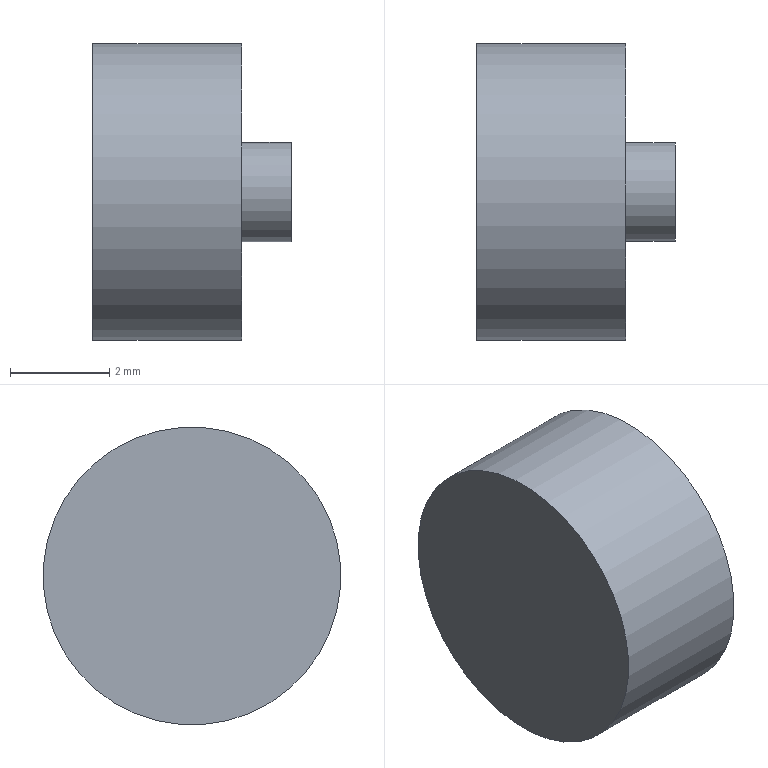Component | NX | LED_LIGHT | 1 solid | 5 faces | box 4 x 6 x 6 mm | volume 88 mm3 | plane 3 | cylinder 2 | commonest cylinder face diameters 6 x1 2 x1
STEP:
#1=CARTESIAN_POINT('',(0.,0.,0.));
#2=DIRECTION('',(0.,0.,1.));
#3=DIRECTION('',(1.,0.,0.));
#4=AXIS2_PLACEMENT_3D('',#1,#2,#3);
#5=CARTESIAN_POINT('',(-14.,-13.074,5.433));
#6=VERTEX_POINT('',#5);
#7=CARTESIAN_POINT('',(-14.,-10.301,6.579));
#8=DIRECTION('',(1.,0.,0.));
#9=DIRECTION('',(0.,-0.9242,-0.3818));
#10=AXIS2_PLACEMENT_3D('',#7,#8,#9);
#11=CIRCLE('',#10,3.);
#12=CARTESIAN_POINT('',(-14.,-10.301,6.579));
#13=DIRECTION('',(1.,0.,0.));
#14=DIRECTION('',(0.,0.9242,0.3818));
#15=AXIS2_PLACEMENT_3D('',#12,#13,#14);
#16=CYLINDRICAL_SURFACE('',#15,3.);
#17=CARTESIAN_POINT('',(3.142,0.));
#18=DIRECTION('',(1.,0.));
#19=VECTOR('',#18,1.);
#20=LINE('',#17,#19);
#21=(GEOMETRIC_REPRESENTATION_CONTEXT(2)PARAMETRIC_REPRESENTATION_CONTEXT()REPRESENTATION_CONTEXT('',''));
#22=DEFINITIONAL_REPRESENTATION('',(#20),#21);
#23=PCURVE('',#16,#22);
#24=CARTESIAN_POINT('',(-14.,-10.301,6.579));
#25=DIRECTION('',(1.,0.,0.));
#26=DIRECTION('',(0.,0.9242,0.3818));
#27=AXIS2_PLACEMENT_3D('',#24,#25,#26);
#28=PLANE('',#27);
#29=CARTESIAN_POINT('',(0.,0.));
#30=DIRECTION('',(-1.,0.));
#31=AXIS2_PLACEMENT_2D('',#29,#30);
#32=CIRCLE('',#31,3.);
#33=(GEOMETRIC_REPRESENTATION_CONTEXT(2)PARAMETRIC_REPRESENTATION_CONTEXT()REPRESENTATION_CONTEXT('',''));
#34=DEFINITIONAL_REPRESENTATION('',(#32),#33);
#35=PCURVE('',#28,#34);
#36=SURFACE_CURVE('',#11,(#23,#35),.PCURVE_S1.);
#37=EDGE_CURVE('',#6,#6,#36,.T.);
#38=ORIENTED_EDGE('',*,*,#37,.T.);
#39=CARTESIAN_POINT('',(-11.,-13.074,5.433));
#40=VERTEX_POINT('',#39);
#41=CARTESIAN_POINT('',(-14.,-13.074,5.433));
#42=CARTESIAN_POINT('',(-11.,-13.074,5.433));
#43=B_SPLINE_CURVE_WITH_KNOTS('',1,(#41,#42),.UNSPECIFIED.,.F.,.F.,(2,2),(0.,3.),.PIECEWISE_BEZIER_KNOTS.);
#44=CARTESIAN_POINT('',(9.425,0.));
#45=DIRECTION('',(0.,1.));
#46=VECTOR('',#45,1.);
#47=LINE('',#44,#46);
#48=(GEOMETRIC_REPRESENTATION_CONTEXT(2)PARAMETRIC_REPRESENTATION_CONTEXT()REPRESENTATION_CONTEXT('',''));
#49=DEFINITIONAL_REPRESENTATION('',(#47),#48);
#50=PCURVE('',#16,#49);
#51=CARTESIAN_POINT('',(3.142,0.));
#52=DIRECTION('',(0.,1.));
#53=VECTOR('',#52,1.);
#54=LINE('',#51,#53);
#55=(GEOMETRIC_REPRESENTATION_CONTEXT(2)PARAMETRIC_REPRESENTATION_CONTEXT()REPRESENTATION_CONTEXT('',''));
#56=DEFINITIONAL_REPRESENTATION('',(#54),#55);
#57=PCURVE('',#16,#56);
#58=SEAM_CURVE('',#43,(#50,#57),.PCURVE_S1.);
#59=EDGE_CURVE('',#6,#40,#58,.T.);
#60=ORIENTED_EDGE('',*,*,#59,.T.);
#61=CARTESIAN_POINT('',(-11.,-10.301,6.579));
#62=DIRECTION('',(1.,0.,0.));
#63=DIRECTION('',(0.,-0.9242,-0.3818));
#64=AXIS2_PLACEMENT_3D('',#61,#62,#63);
#65=CIRCLE('',#64,3.);
#66=CARTESIAN_POINT('',(3.142,3.));
#67=DIRECTION('',(1.,0.));
#68=VECTOR('',#67,1.);
#69=LINE('',#66,#68);
#70=(GEOMETRIC_REPRESENTATION_CONTEXT(2)PARAMETRIC_REPRESENTATION_CONTEXT()REPRESENTATION_CONTEXT('',''));
#71=DEFINITIONAL_REPRESENTATION('',(#69),#70);
#72=PCURVE('',#16,#71);
#73=CARTESIAN_POINT('',(-11.,-10.301,6.579));
#74=DIRECTION('',(1.,0.,0.));
#75=DIRECTION('',(0.,0.9242,0.3818));
#76=AXIS2_PLACEMENT_3D('',#73,#74,#75);
#77=PLANE('',#76);
#78=CARTESIAN_POINT('',(0.,0.));
#79=DIRECTION('',(-1.,0.));
#80=AXIS2_PLACEMENT_2D('',#78,#79);
#81=CIRCLE('',#80,3.);
#82=(GEOMETRIC_REPRESENTATION_CONTEXT(2)PARAMETRIC_REPRESENTATION_CONTEXT()REPRESENTATION_CONTEXT('',''));
#83=DEFINITIONAL_REPRESENTATION('',(#81),#82);
#84=PCURVE('',#77,#83);
#85=SURFACE_CURVE('',#65,(#72,#84),.PCURVE_S1.);
#86=EDGE_CURVE('',#40,#40,#85,.T.);
#87=ORIENTED_EDGE('',*,*,#86,.F.);
#88=ORIENTED_EDGE('',*,*,#59,.F.);
#89=EDGE_LOOP('',(#38,#60,#87,#88));
#90=FACE_BOUND('',#89,.T.);
#91=ADVANCED_FACE('',(#90),#16,.T.);
#92=ORIENTED_EDGE('',*,*,#37,.F.);
#93=EDGE_LOOP('',(#92));
#94=FACE_BOUND('',#93,.T.);
#95=ADVANCED_FACE('',(#94),#28,.F.);
#96=CARTESIAN_POINT('',(-11.,-11.225,6.197));
#97=VERTEX_POINT('',#96);
#98=CARTESIAN_POINT('',(-11.,-10.301,6.579));
#99=DIRECTION('',(-1.,0.,0.));
#100=DIRECTION('',(0.,-0.9242,-0.3818));
#101=AXIS2_PLACEMENT_3D('',#98,#99,#100);
#102=CIRCLE('',#101,1.);
#103=CARTESIAN_POINT('',(-1.,-0.));
#104=CARTESIAN_POINT('',(-1.,1.732));
#105=CARTESIAN_POINT('',(0.5,0.866));
#106=CARTESIAN_POINT('',(2.,0.));
#107=CARTESIAN_POINT('',(0.5,-0.866));
#108=CARTESIAN_POINT('',(-1.,-1.732));
#109=CARTESIAN_POINT('',(-1.,-0.));
#110=(BOUNDED_CURVE()B_SPLINE_CURVE(2,(#103,#104,#105,#106,#107,#108,#109),.UNSPECIFIED.,.T.,.F.)B_SPLINE_CURVE_WITH_KNOTS((1,2,2,2,2,1),(-2.094,0.,2.094,4.189,6.283,8.378),.UNSPECIFIED.)CURVE()GEOMETRIC_REPRESENTATION_ITEM()RATIONAL_B_SPLINE_CURVE((1.,0.5,1.,0.5,1.,0.5,1.))REPRESENTATION_ITEM(''));
#111=(GEOMETRIC_REPRESENTATION_CONTEXT(2)PARAMETRIC_REPRESENTATION_CONTEXT()REPRESENTATION_CONTEXT('',''));
#112=DEFINITIONAL_REPRESENTATION('',(#110),#111);
#113=PCURVE('',#77,#112);
#114=CARTESIAN_POINT('',(-10.,-10.301,6.579));
#115=DIRECTION('',(-1.,0.,0.));
#116=DIRECTION('',(0.,-0.9242,-0.3818));
#117=AXIS2_PLACEMENT_3D('',#114,#115,#116);
#118=CYLINDRICAL_SURFACE('',#117,1.);
#119=CARTESIAN_POINT('',(0.,1.));
#120=DIRECTION('',(1.,0.));
#121=VECTOR('',#120,1.);
#122=LINE('',#119,#121);
#123=(GEOMETRIC_REPRESENTATION_CONTEXT(2)PARAMETRIC_REPRESENTATION_CONTEXT()REPRESENTATION_CONTEXT('',''));
#124=DEFINITIONAL_REPRESENTATION('',(#122),#123);
#125=PCURVE('',#118,#124);
#126=SURFACE_CURVE('',#102,(#113,#125),.PCURVE_S1.);
#127=EDGE_CURVE('',#97,#97,#126,.T.);
#128=ORIENTED_EDGE('',*,*,#127,.T.);
#129=EDGE_LOOP('',(#128));
#130=FACE_BOUND('',#129,.T.);
#131=ORIENTED_EDGE('',*,*,#86,.T.);
#132=EDGE_LOOP('',(#131));
#133=FACE_BOUND('',#132,.T.);
#134=ADVANCED_FACE('',(#130,#133),#77,.T.);
#135=CARTESIAN_POINT('',(-10.,-11.225,6.197));
#136=VERTEX_POINT('',#135);
#137=CARTESIAN_POINT('',(-10.,-10.301,6.579));
#138=DIRECTION('',(-1.,0.,0.));
#139=DIRECTION('',(0.,-0.9242,-0.3818));
#140=AXIS2_PLACEMENT_3D('',#137,#138,#139);
#141=CIRCLE('',#140,1.);
#142=CARTESIAN_POINT('',(0.,0.));
#143=DIRECTION('',(1.,0.));
#144=VECTOR('',#143,1.);
#145=LINE('',#142,#144);
#146=(GEOMETRIC_REPRESENTATION_CONTEXT(2)PARAMETRIC_REPRESENTATION_CONTEXT()REPRESENTATION_CONTEXT('',''));
#147=DEFINITIONAL_REPRESENTATION('',(#145),#146);
#148=PCURVE('',#118,#147);
#149=CARTESIAN_POINT('',(-10.,-10.301,6.579));
#150=DIRECTION('',(-1.,0.,0.));
#151=DIRECTION('',(0.,-0.9242,-0.3818));
#152=AXIS2_PLACEMENT_3D('',#149,#150,#151);
#153=PLANE('',#152);
#154=CARTESIAN_POINT('',(0.,0.));
#155=DIRECTION('',(1.,-0.));
#156=AXIS2_PLACEMENT_2D('',#154,#155);
#157=CIRCLE('',#156,1.);
#158=(GEOMETRIC_REPRESENTATION_CONTEXT(2)PARAMETRIC_REPRESENTATION_CONTEXT()REPRESENTATION_CONTEXT('',''));
#159=DEFINITIONAL_REPRESENTATION('',(#157),#158);
#160=PCURVE('',#153,#159);
#161=SURFACE_CURVE('',#141,(#148,#160),.PCURVE_S1.);
#162=EDGE_CURVE('',#136,#136,#161,.T.);
#163=ORIENTED_EDGE('',*,*,#162,.T.);
#164=CARTESIAN_POINT('',(-10.,-11.225,6.197));
#165=CARTESIAN_POINT('',(-11.,-11.225,6.197));
#166=B_SPLINE_CURVE_WITH_KNOTS('',1,(#164,#165),.UNSPECIFIED.,.F.,.F.,(2,2),(0.,1.),.PIECEWISE_BEZIER_KNOTS.);
#167=CARTESIAN_POINT('',(6.283,0.));
#168=DIRECTION('',(0.,1.));
#169=VECTOR('',#168,1.);
#170=LINE('',#167,#169);
#171=(GEOMETRIC_REPRESENTATION_CONTEXT(2)PARAMETRIC_REPRESENTATION_CONTEXT()REPRESENTATION_CONTEXT('',''));
#172=DEFINITIONAL_REPRESENTATION('',(#170),#171);
#173=PCURVE('',#118,#172);
#174=CARTESIAN_POINT('',(0.,0.));
#175=DIRECTION('',(0.,1.));
#176=VECTOR('',#175,1.);
#177=LINE('',#174,#176);
#178=(GEOMETRIC_REPRESENTATION_CONTEXT(2)PARAMETRIC_REPRESENTATION_CONTEXT()REPRESENTATION_CONTEXT('',''));
#179=DEFINITIONAL_REPRESENTATION('',(#177),#178);
#180=PCURVE('',#118,#179);
#181=SEAM_CURVE('',#166,(#173,#180),.PCURVE_S1.);
#182=EDGE_CURVE('',#136,#97,#181,.T.);
#183=ORIENTED_EDGE('',*,*,#182,.T.);
#184=ORIENTED_EDGE('',*,*,#127,.F.);
#185=ORIENTED_EDGE('',*,*,#182,.F.);
#186=EDGE_LOOP('',(#163,#183,#184,#185));
#187=FACE_BOUND('',#186,.T.);
#188=ADVANCED_FACE('',(#187),#118,.T.);
#189=ORIENTED_EDGE('',*,*,#162,.F.);
#190=EDGE_LOOP('',(#189));
#191=FACE_BOUND('',#190,.T.);
#192=ADVANCED_FACE('',(#191),#153,.F.);
#193=CLOSED_SHELL('',(#91,#95,#134,#188,#192));
#194=MANIFOLD_SOLID_BREP('',#193);
#195=(LENGTH_UNIT()NAMED_UNIT(*)SI_UNIT(.MILLI.,.METRE.));
#196=UNCERTAINTY_MEASURE_WITH_UNIT(LENGTH_MEASURE(0.00001),#195,'','');
#197=(NAMED_UNIT(*)PLANE_ANGLE_UNIT()SI_UNIT($,.RADIAN.));
#198=(NAMED_UNIT(*)SI_UNIT($,.STERADIAN.)SOLID_ANGLE_UNIT());
#199=(GEOMETRIC_REPRESENTATION_CONTEXT(3)GLOBAL_UNCERTAINTY_ASSIGNED_CONTEXT((#196))GLOBAL_UNIT_ASSIGNED_CONTEXT((#195,#197,#198))REPRESENTATION_CONTEXT('',''));
#200=ADVANCED_BREP_SHAPE_REPRESENTATION('',(#4,#194),#199);